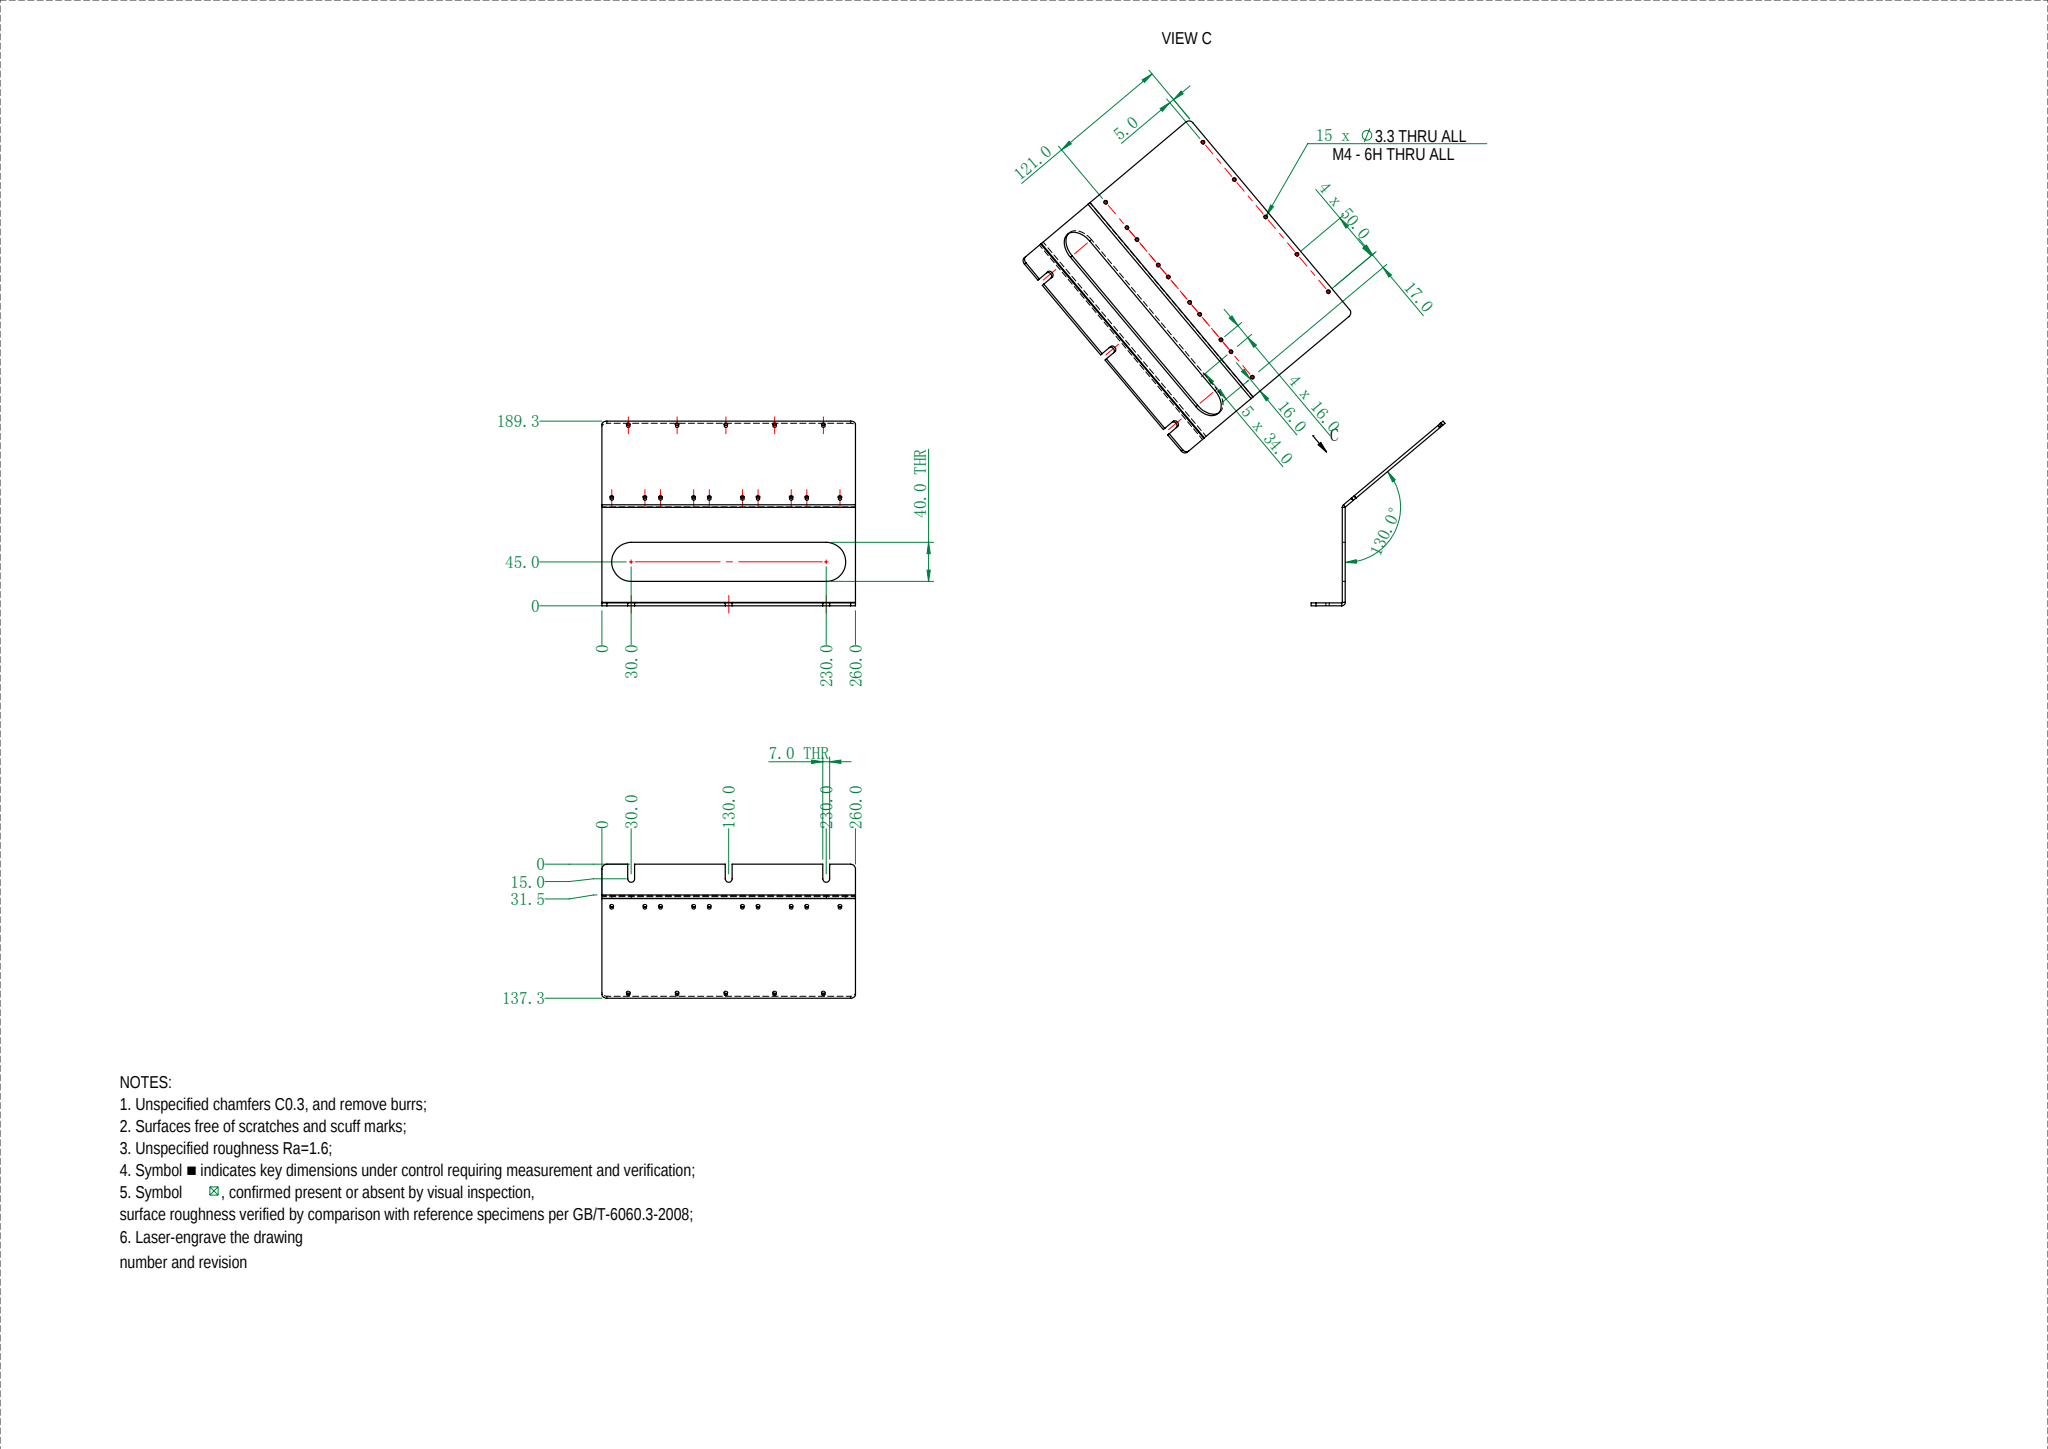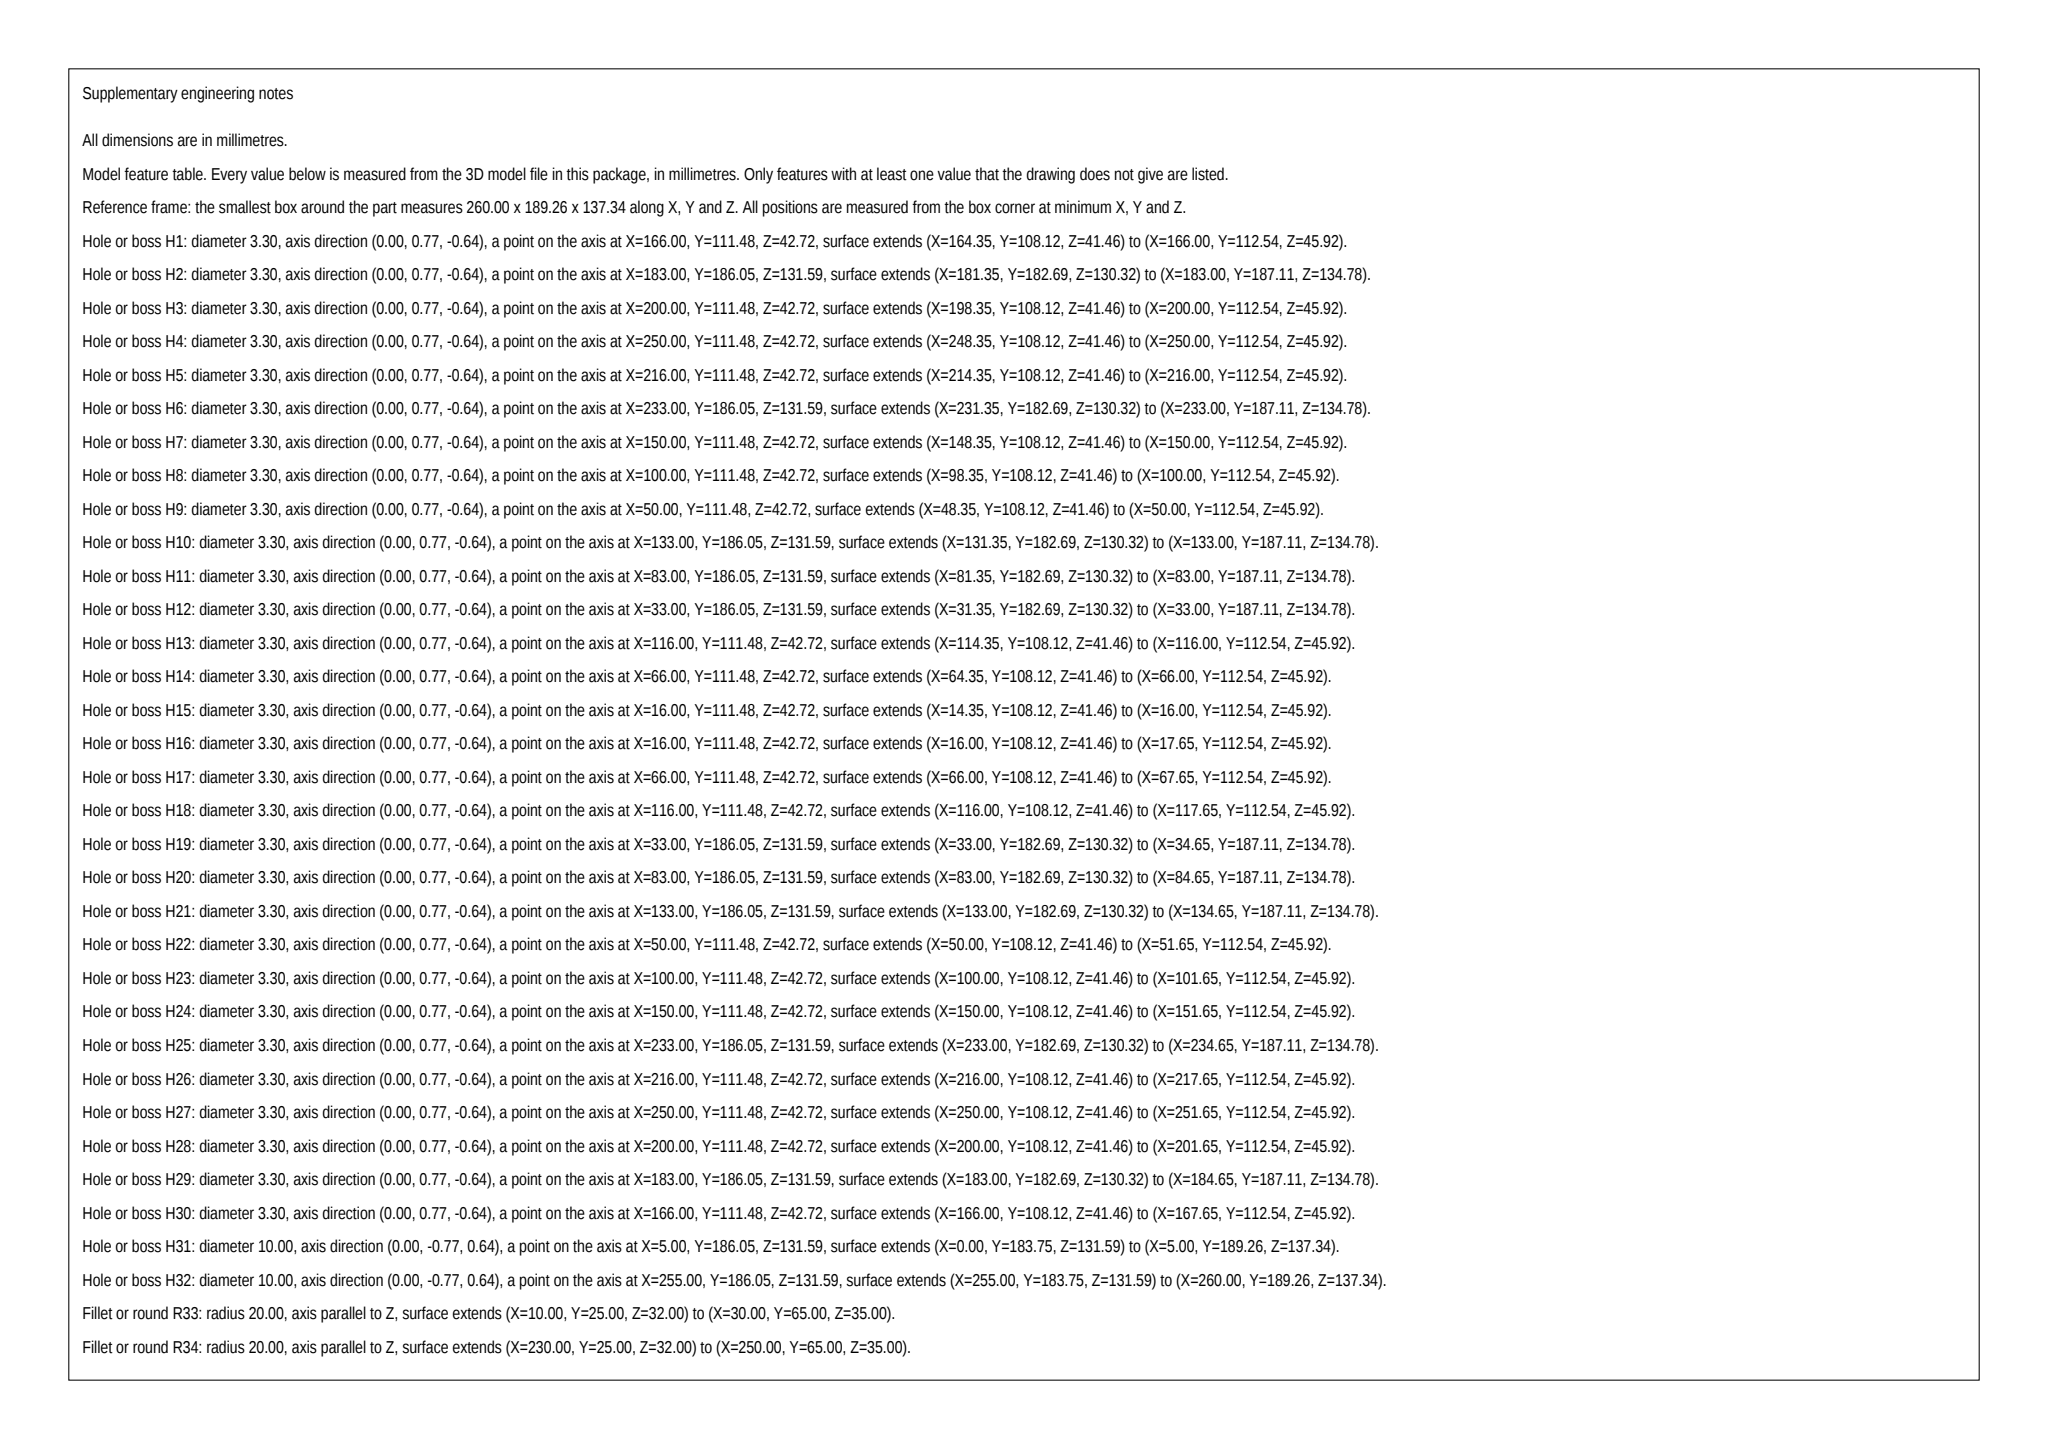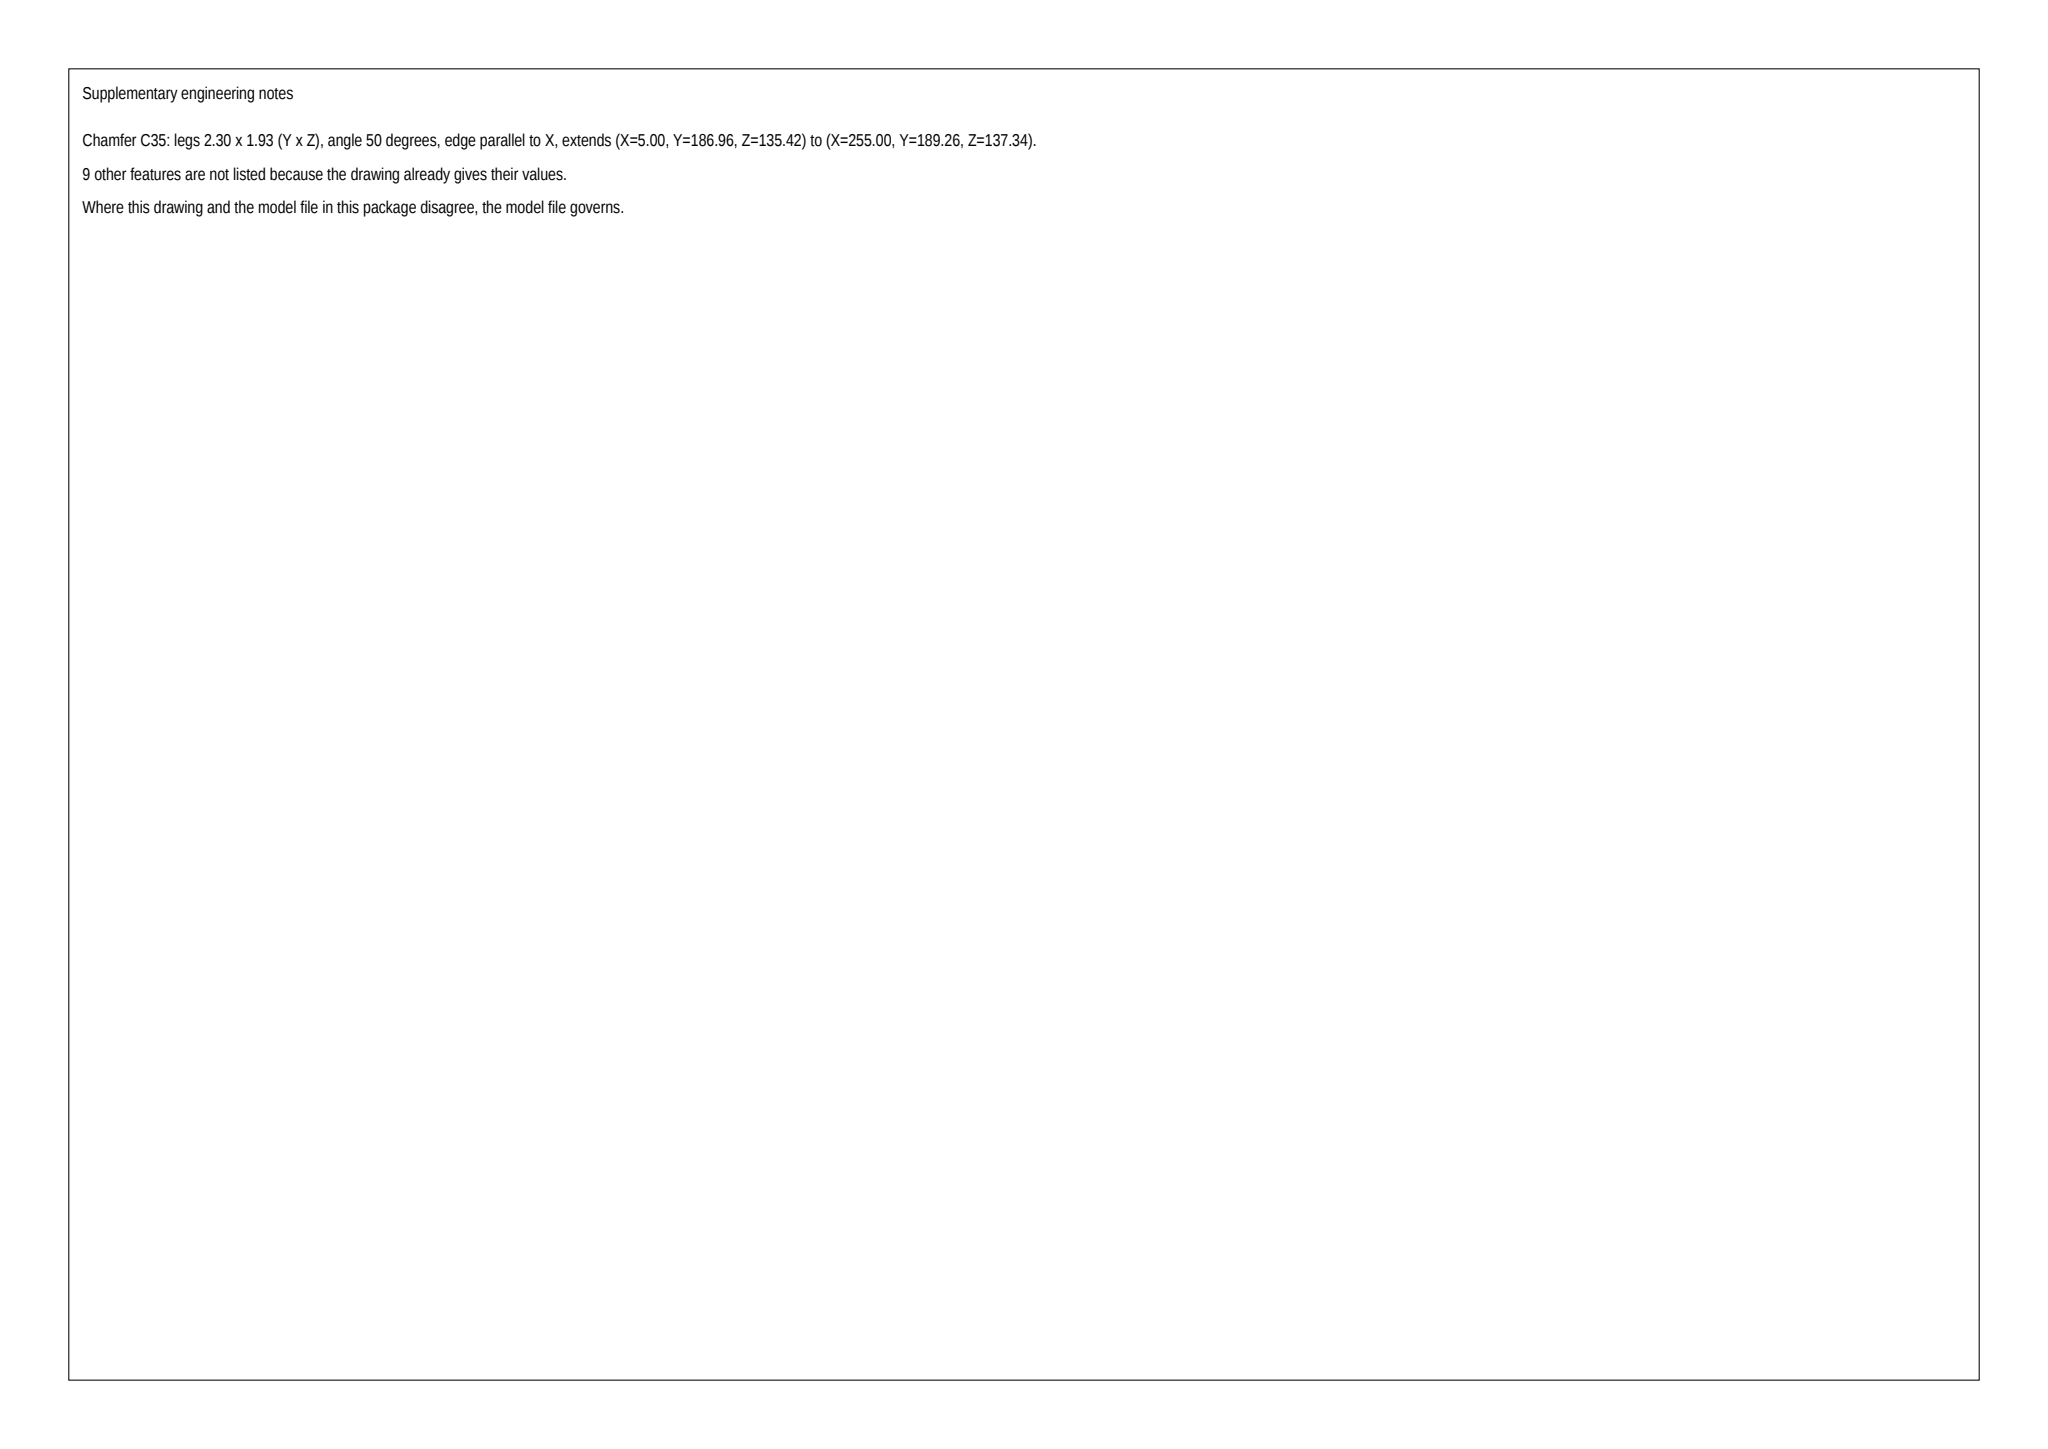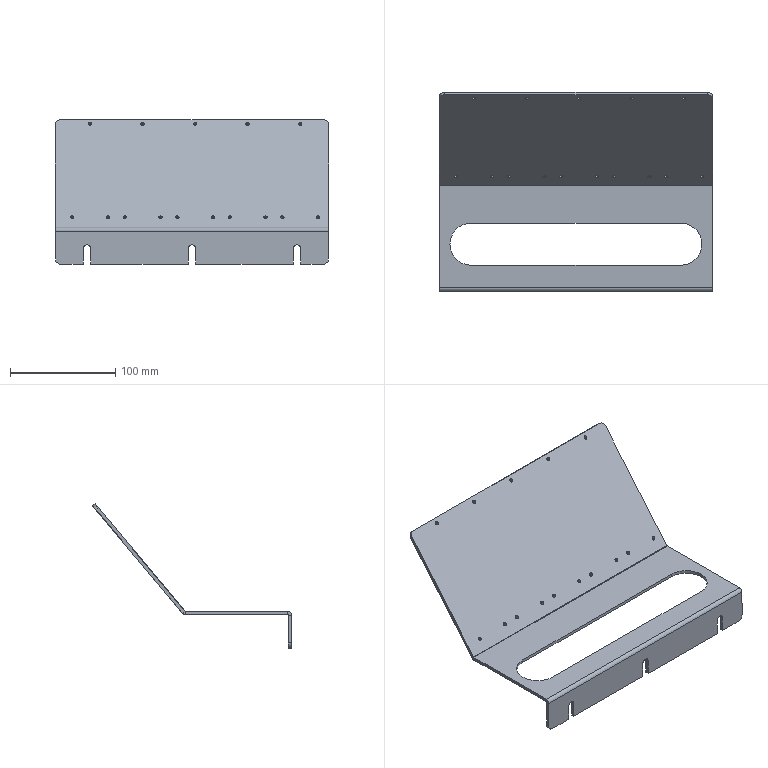Part | SolidWorks | mm | 1 solid | 76 faces | box 260 x 189.26 x 137.34 mm | volume 179005 mm3 | cylinder 47 | plane 29 | commonest cylinder face diameters 3.3 x30 7 x8 10 x4 40 x3 1 x2
Drawing notes:
OBROUND SLOT 40 WIDE x 240 OA, R20 ENDS; END CL 30 & 230 FROM LH EDGE, THRU | from the solid: cyl dia40 axis z at (30,45) & (230,45), len 3.0 = thru 3 thk wall; ends 200 apart, 240 OA
3X NOTCH 7 WIDE x 15 DP, R3.5 END, CL 30, 130, 230 FROM LH EDGE | from the solid: cyl dia7 axis y at x=30/130/230, z=15, len 3.0; x-planes 26.5/33.5, 126.5/133.5, 226.5/233.5
3 THK; BEND TANGENTS 31.5 FROM FRONT EDGE & 100.85 FROM BTM, R0.5 INSIDE | from the solid: bend axis cyls (y=3.5,z=31.5) & (y=100.85,z=35.5) len 260; y-planes 0/3.0, z-planes 32.0/35.0
UPPER BEND: UPPER PANEL AT 50.0° TO BASE PANEL (INTERIOR ANGLE 130.0°); BEND LINE 100.85 FROM FRONT FLANGE FACE, R0.5 INSIDE, 3.0 THK | from the solid: cylinders dia 1.0 and 7.0, axis x, at (y=100.85, z=35.5), length 260 (inside R0.5 / outside R3.5 bend) together with bbox 189.259 (Y) x 137.344 (Z) -> panel rises 50.0deg from base plane
15 x Ø3.3 THRU IN TILTED UPPER PANEL: LOWER ROW OF 10 HOLES AT 42.72 AND UPPER ROW OF 5 HOLES AT 131.59, BOTH MEASURED FROM NOTCHED FRONT-FLANGE EDGE (Z0 DATUM) | from the solid: cylinders dia 3.3 axis y at z=42.72 (10 holes) and z=131.59 (5 holes)
HOLE ROWS FROM LH EDGE (X0): UPPER ROW FIRST HOLE 33.0, THEN 4 x 50.0; LOWER ROW FIRST HOLE 16.0, THEN 34.0/16.0 ALTERNATING TO 250.0 | from the solid: cylinders dia 3.3 axis y at x=33,83,133,183,233 (z=131.59) and x=16,50,66,100,116,150,166,200,216,250 (z=42.72)
15X Ø3.3 THRU ALL (M4-6H): 10 holes on lower face at Z=42.72 from bottom, X = 16, 50, 66, 100, 116, 150, 166, 200, 216, 250 from LH edge (X=0 datum) | from the solid: cylinders dia 3.3 axis y at z=42.72, x = 16,50,66,100,116,150,166,200,216,250
5X Ø3.3 THRU ALL (M4-6H) on upper tilted panel: Z=131.59 from bottom face, X = 33, 83, 133, 183, 233 from LH edge (X=0 datum) | from the solid: cylinders dia 3.3 axis y at z=131.59, x = 33,83,133,183,233
Lower bend 90.0°, R0.5 inside; bend radius centerline at Y=3.5, Z=31.5 from min corner (bottom/front faces at Y=0 and Z=0) | from the solid: cylinders dia 1.0/7.0 axis x at [y 3.5, z 31.5]; axis planes y=0, y=3.0, z=0
Upper bend R0.5 inside; bend radius centerline at Y=100.85, Z=35.5 from min corner | from the solid: cylinders dia 1.0/7.0 axis x at [y 100.85, z 35.5]
Material thickness 3.0; overall envelope 260.0 X x 189.259 Y x 137.344 Z | from the solid: bbox_xyz [260.0, 189.259, 137.344]; axis planes y=0 and y=3.0
MATERIAL THICKNESS 3.0 UNIFORM (parallel faces at Y=0 and Y=3.0 datum) | from the solid: axis_planes y=0.0 and y=3.0; supplementary thickness 3.0
2X BEND R0.5 INSIDE: lower bend radius CL at Y=3.5, Z=31.5; upper bend radius CL at Y=100.85, Z=35.5 (from min corner datum) | from the solid: cylinders dia 1.0 axis x at [null,3.5,31.5] and [null,100.85,35.5]
4X R5.0 CORNER RADII: centers at X=5.0 and X=255.0 from LH edge (X=0), at Z=5.0 (front panel) and Z=131.59 (tilted upper panel) | from the solid: cylinders dia 10.0 axis y at [5.0,null,5.0], [255.0,null,5.0], [5.0,null,131.59], [255.0,null,131.59]
OBROUND SLOT 40.0 WIDE THRU FRONT PANEL: end radii centers X=30.0 and X=230.0 from LH edge (X=0), Y=45.0; thru 3.0 wall | from the solid: cylinders dia 40.0 axis z at [30.0,45.0] and [230.0,45.0], length 3.0
3X NOTCH 7.0 WIDE THRU, R3.5 END: notch end radius centers X=30.0, 130.0, 230.0 from LH edge (X=0) at Z=15.0 from bottom face (Z=0) | from the solid: cylinders dia 7.0 axis y at [30.0,null,15.0], [130.0,null,15.0], [230.0,null,15.0], length 3.0